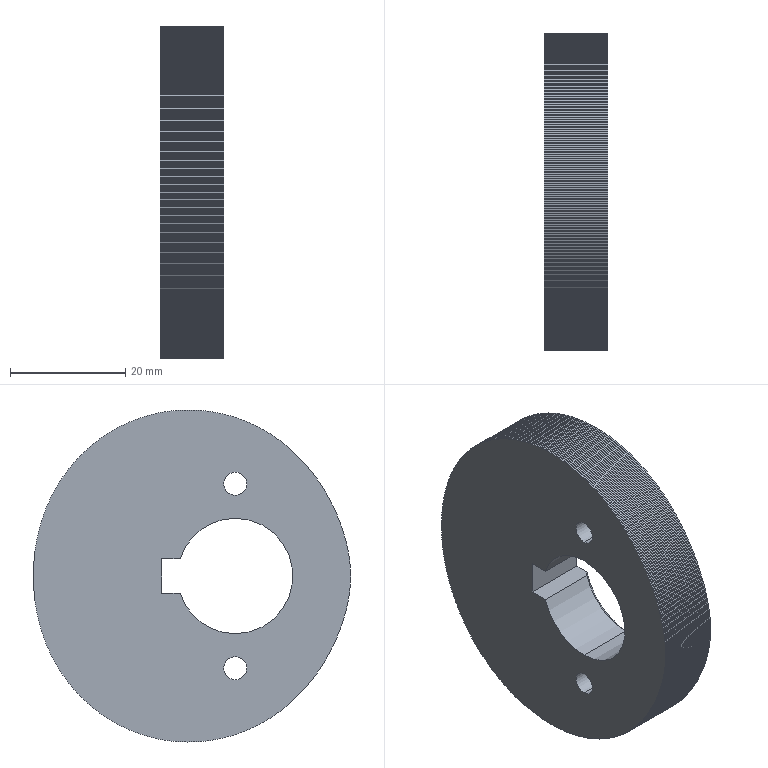Component | SolidWorks | CamGroup3-1_Cam1-1 | 1 solid | 644 faces | volume 23291 mm3 | plane 634 | cylinder 7 | cone 3 | commonest cylinder face diameters 4 x4 20 x3